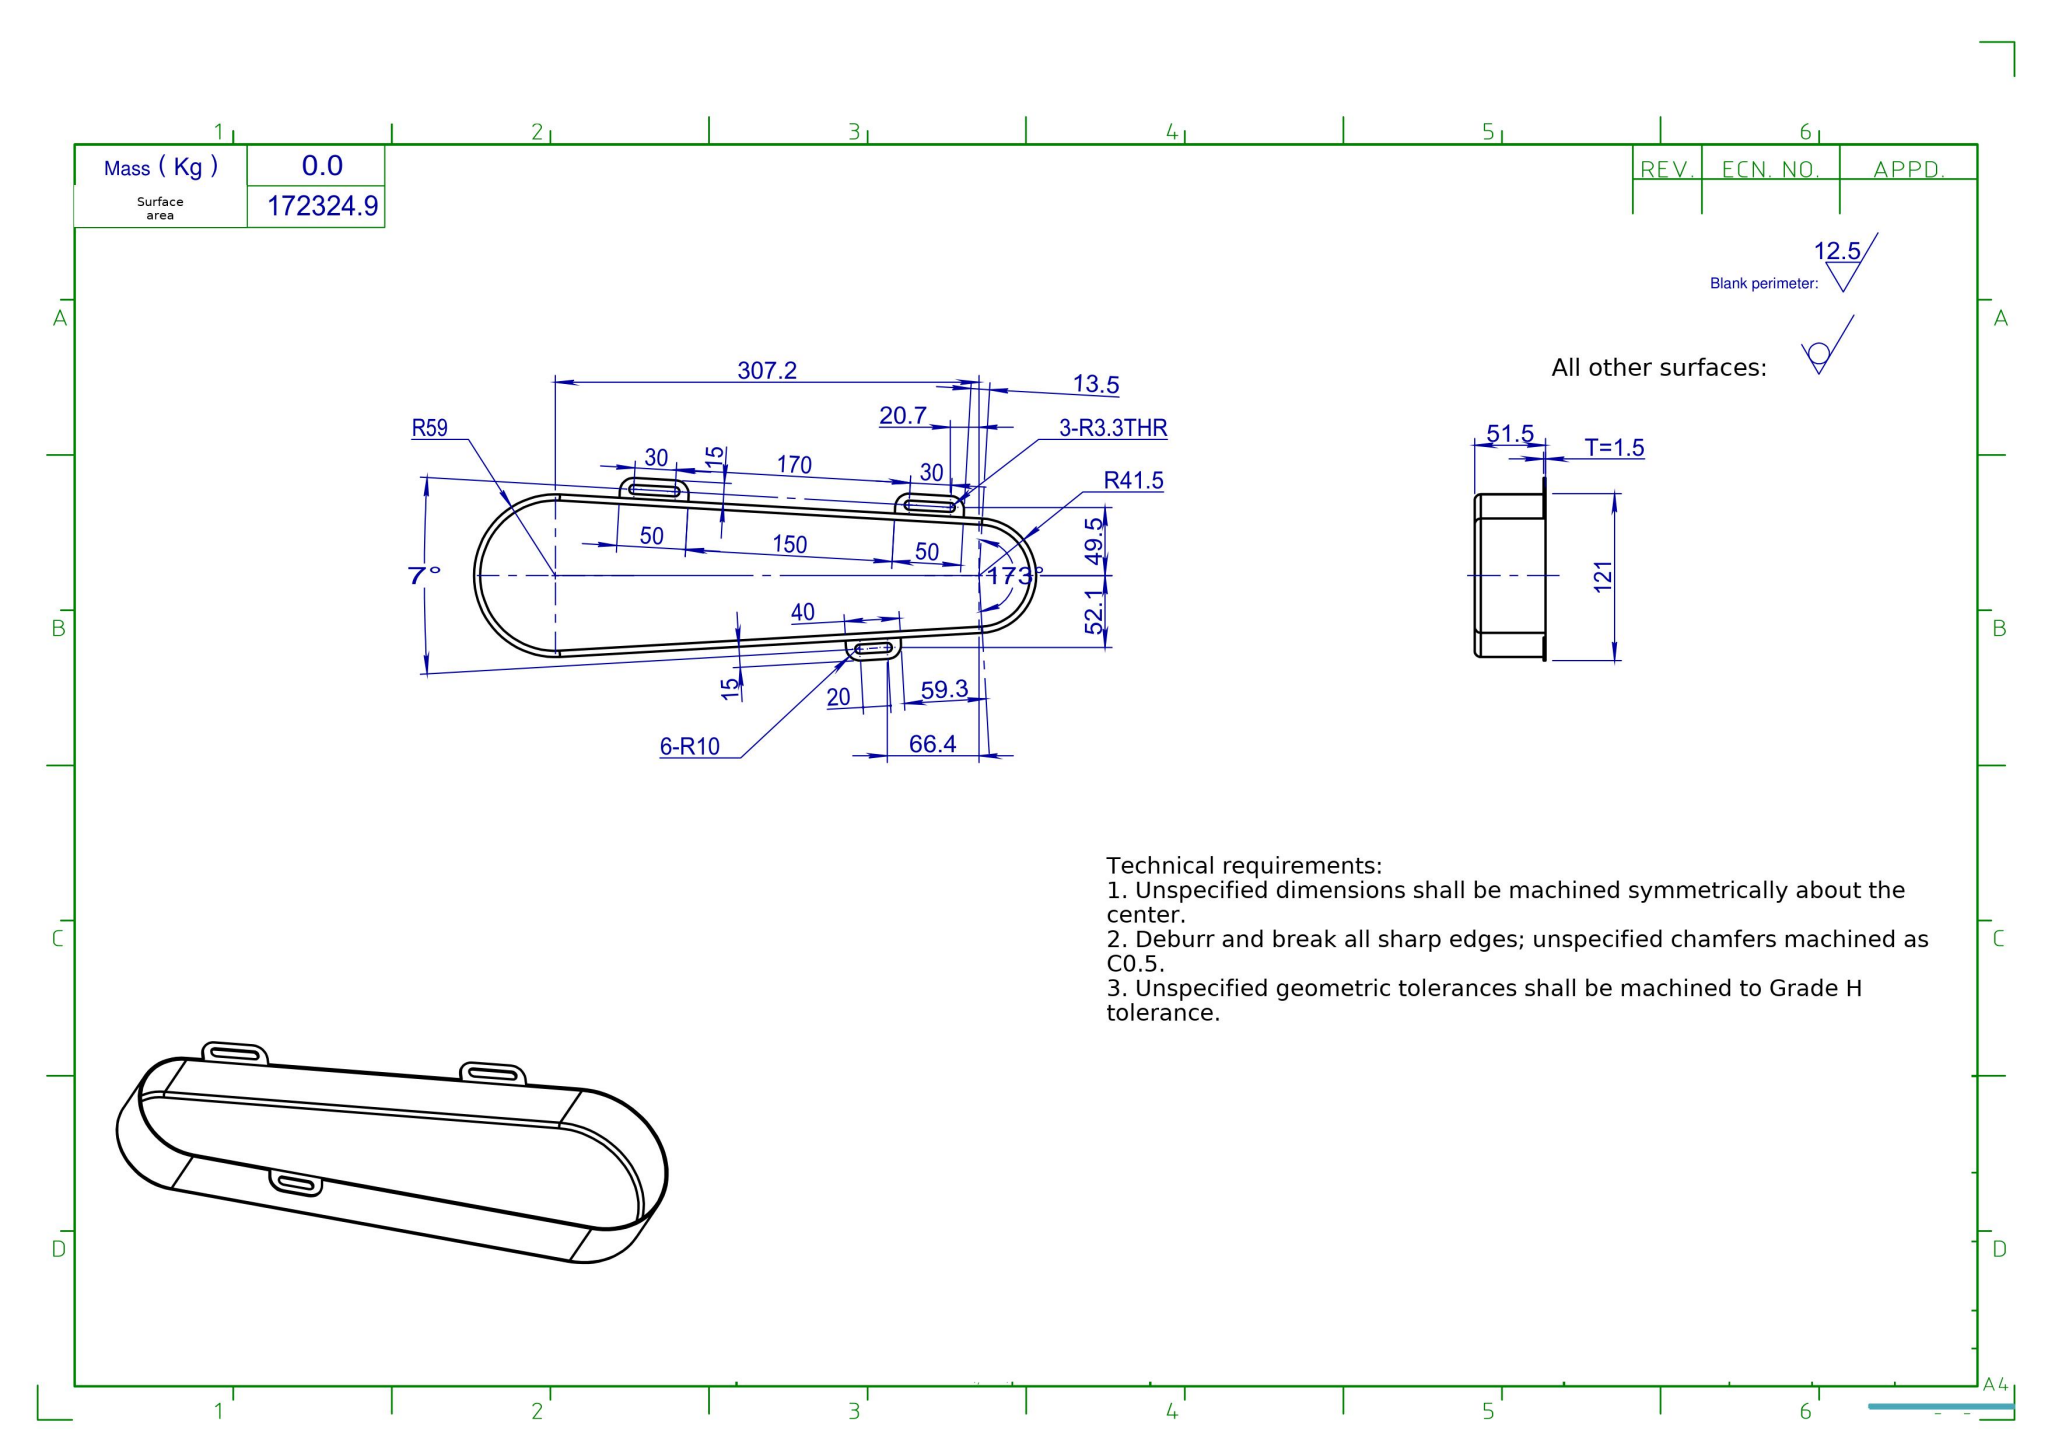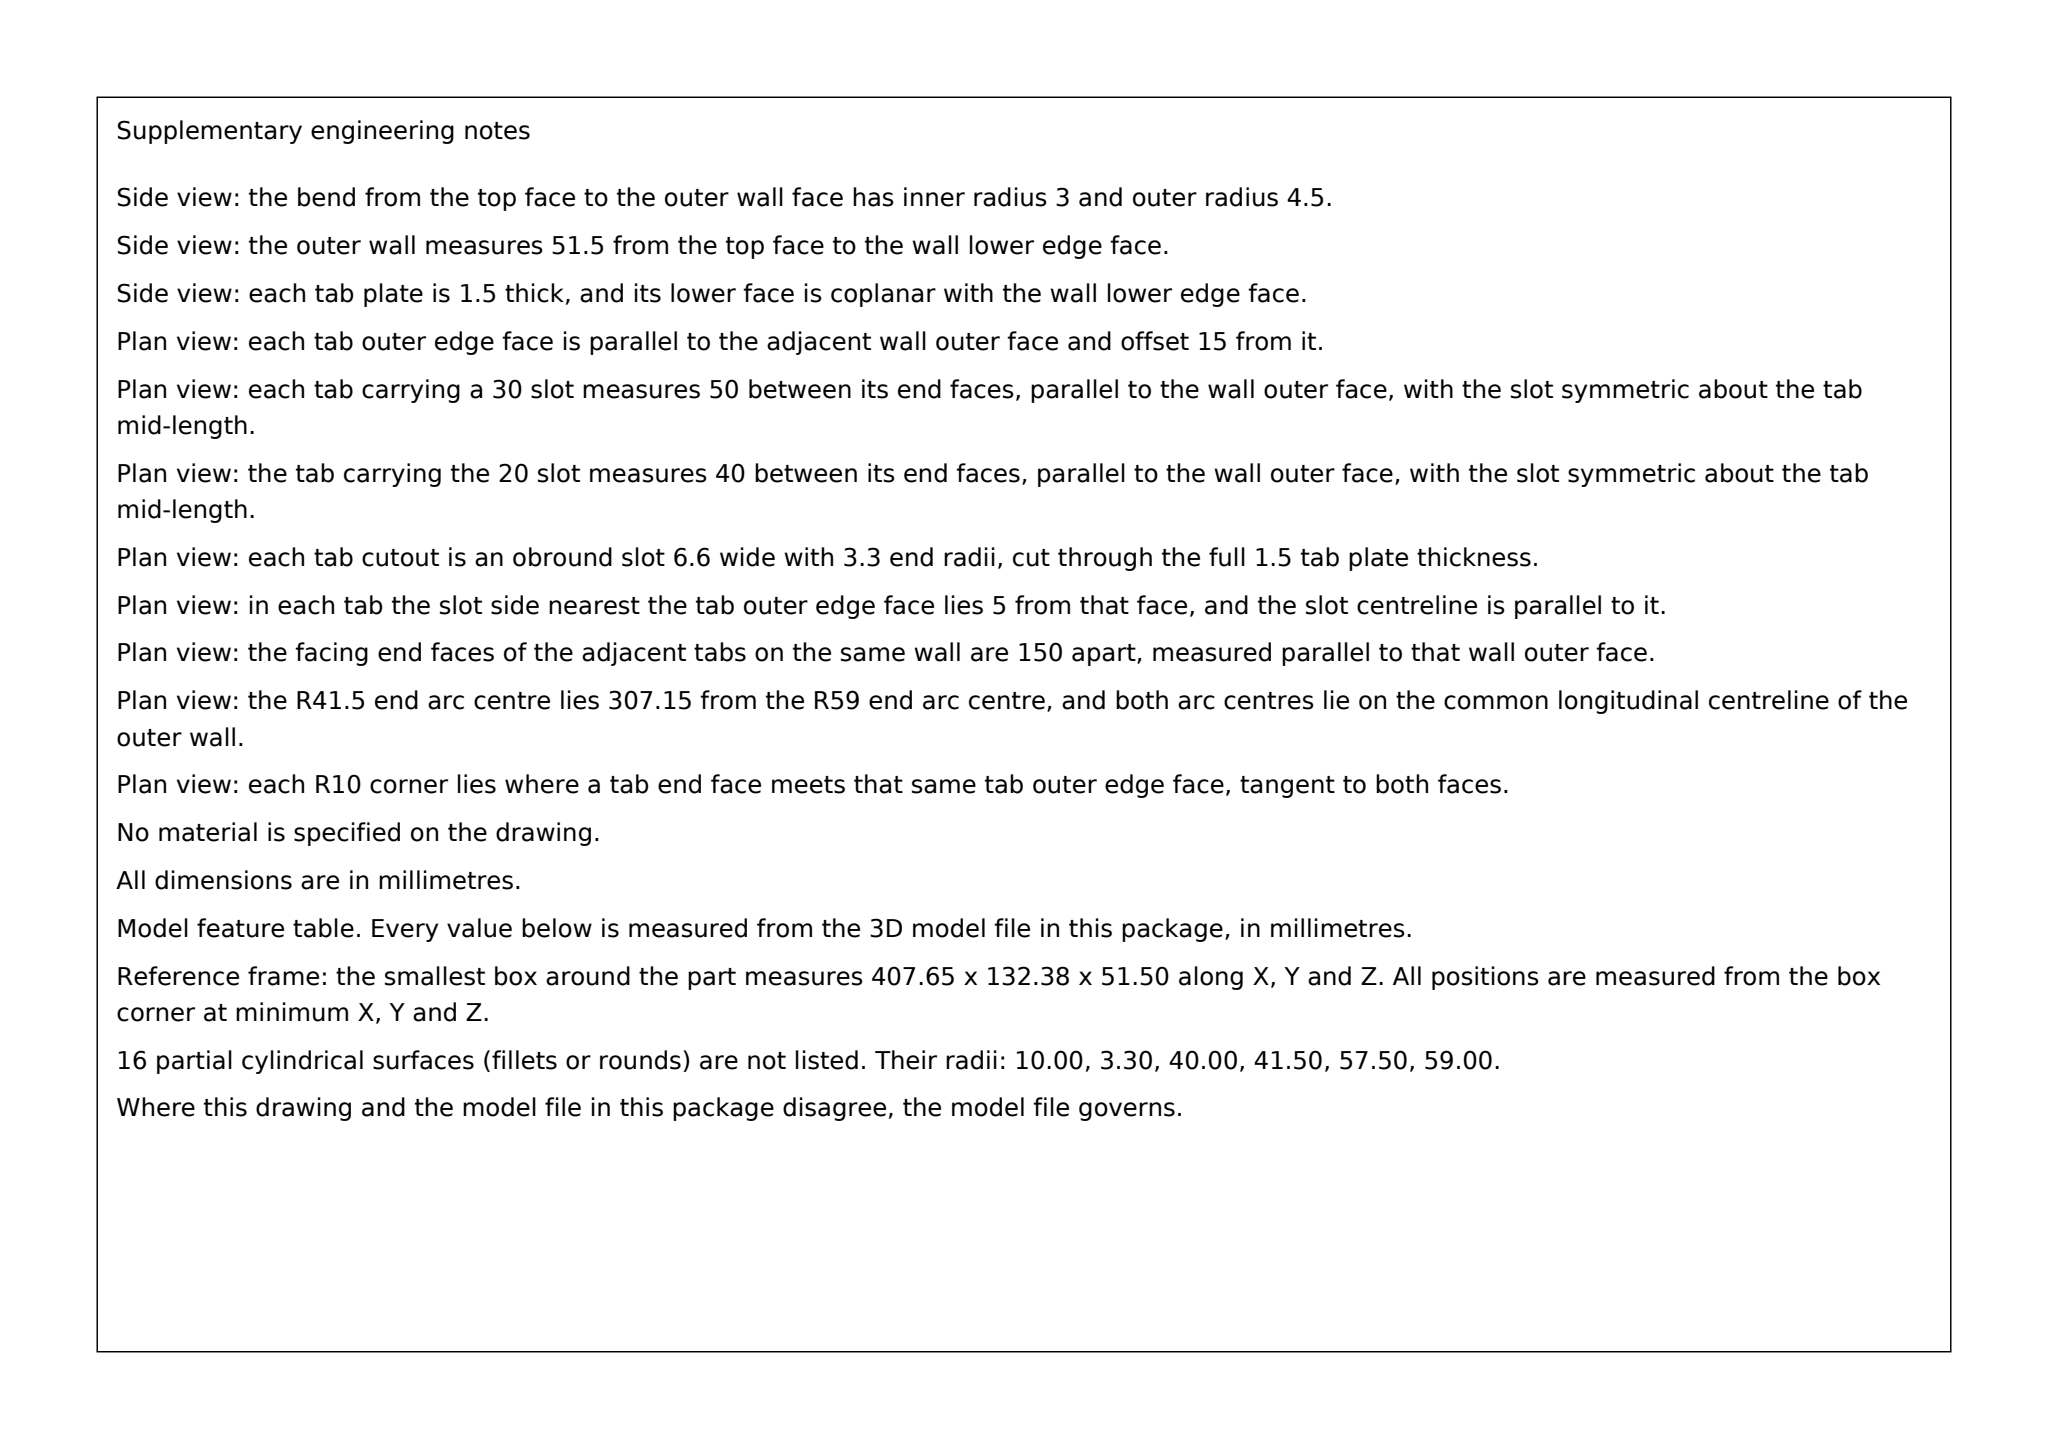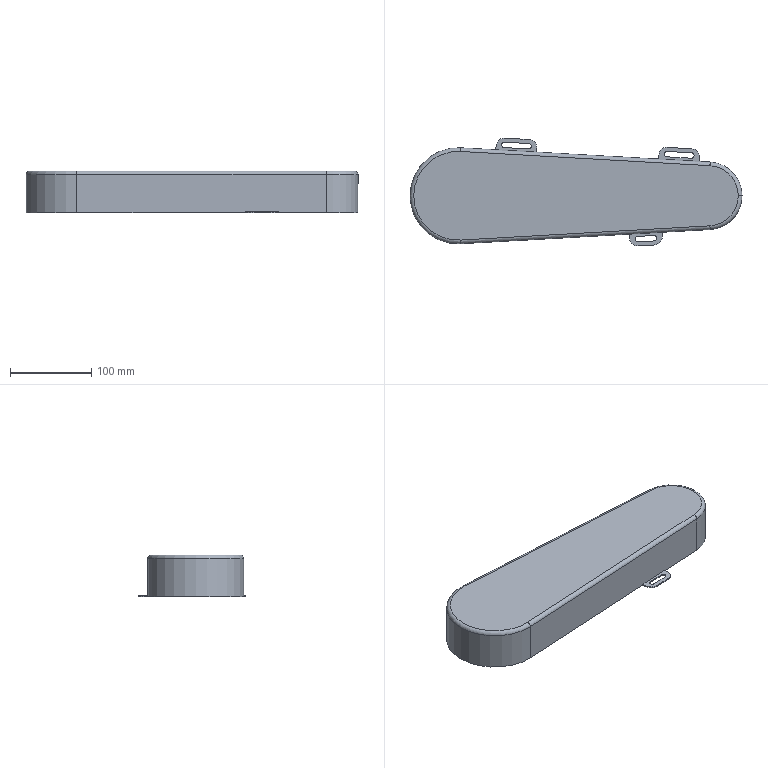Part | SolidWorks | mm | 1 solid | 61 faces | box 407.65 x 132.38 x 51.5 mm | volume 127876 mm3 | plane 28 | cylinder 27 | torus 6 | commonest cylinder face diameters 6.6 x9 20 x8 80 x2 83 x2 9 x2 6 x2 118 x1 115 x1
Drawing notes:
3-R3 AND 3-R4.5 FILLETS AT RAISED SLOT TAB TRANSITIONS | from the solid: fillet_radii: [[3.0,3],[4.5,3]] at the 20.0 dia raised pads with 6.6 slots
UNSPECIFIED FILLETS: R3 | from the solid: smallest modeled fillet radius 3.0 (qty 3)
3-SLOT TABS (20 WIDE, R10) RAISED 1.5 ABOVE SHELL FACE | from the solid: Dia 20 & 6.6 z-cylinders, length 1.5; planes z=0 and z=1.5
INT CAVITY DEPTH 47 FROM BACK FACE; STEP FACE AT 50; T=1.5 | from the solid: Dia 115/118 & 80/83 z-cylinders length 47; planes z=0, 50.0, 51.5
WIDTH ACROSS R59 END = 118 OD (INNER R57.5, WALL T=1.5) | from the solid: Coaxial z-cylinders dia 118 and 115 at (63.86, 63.86)